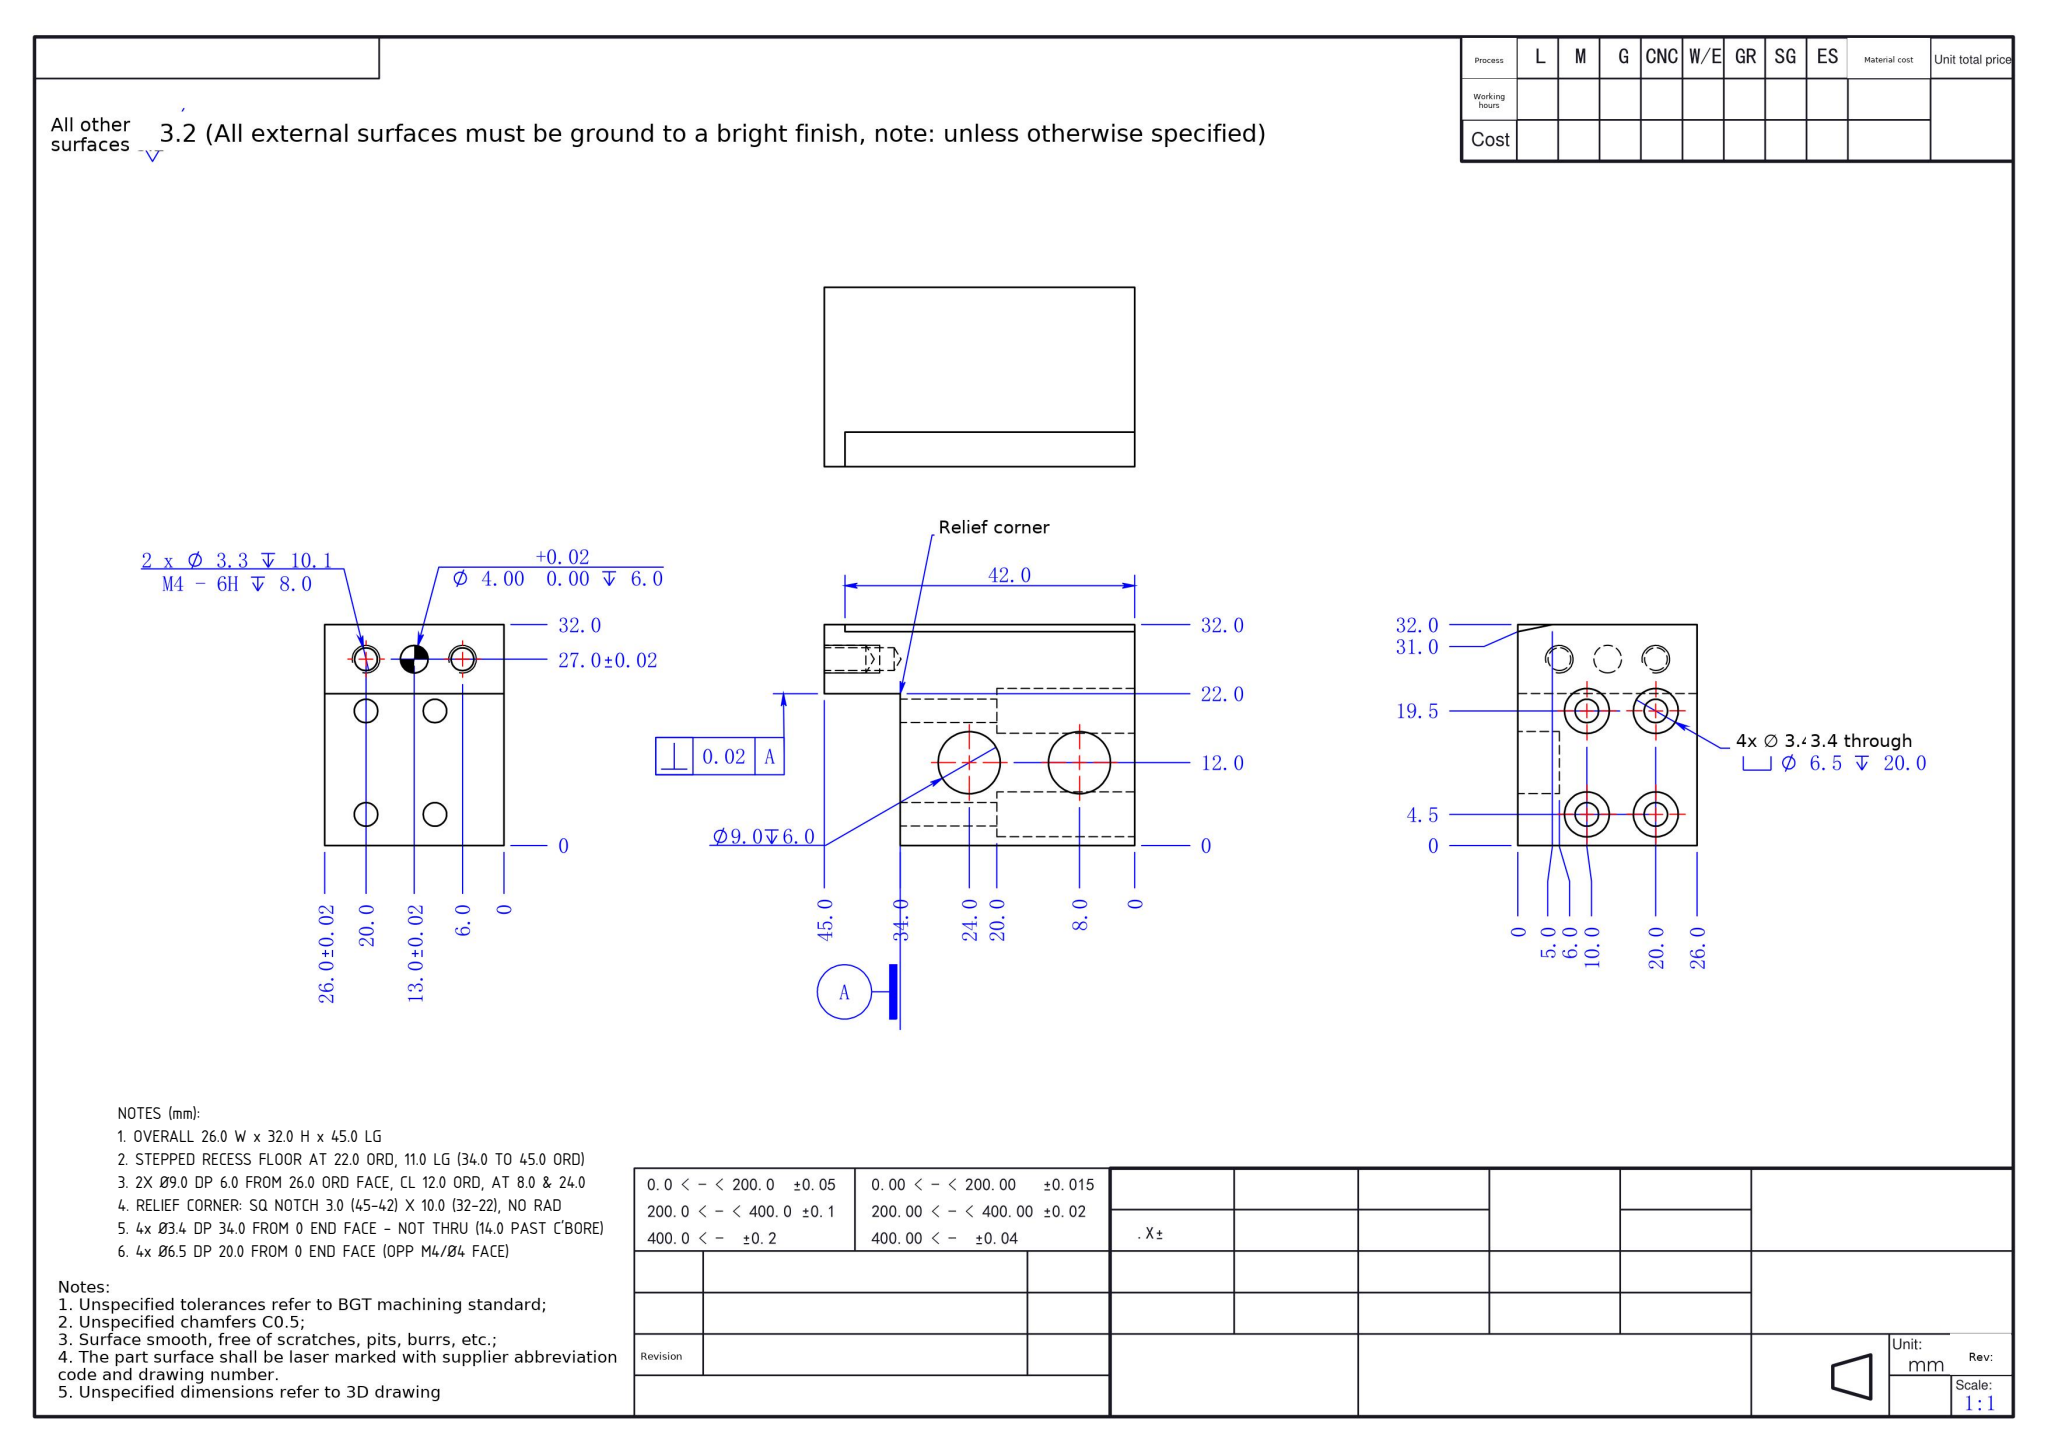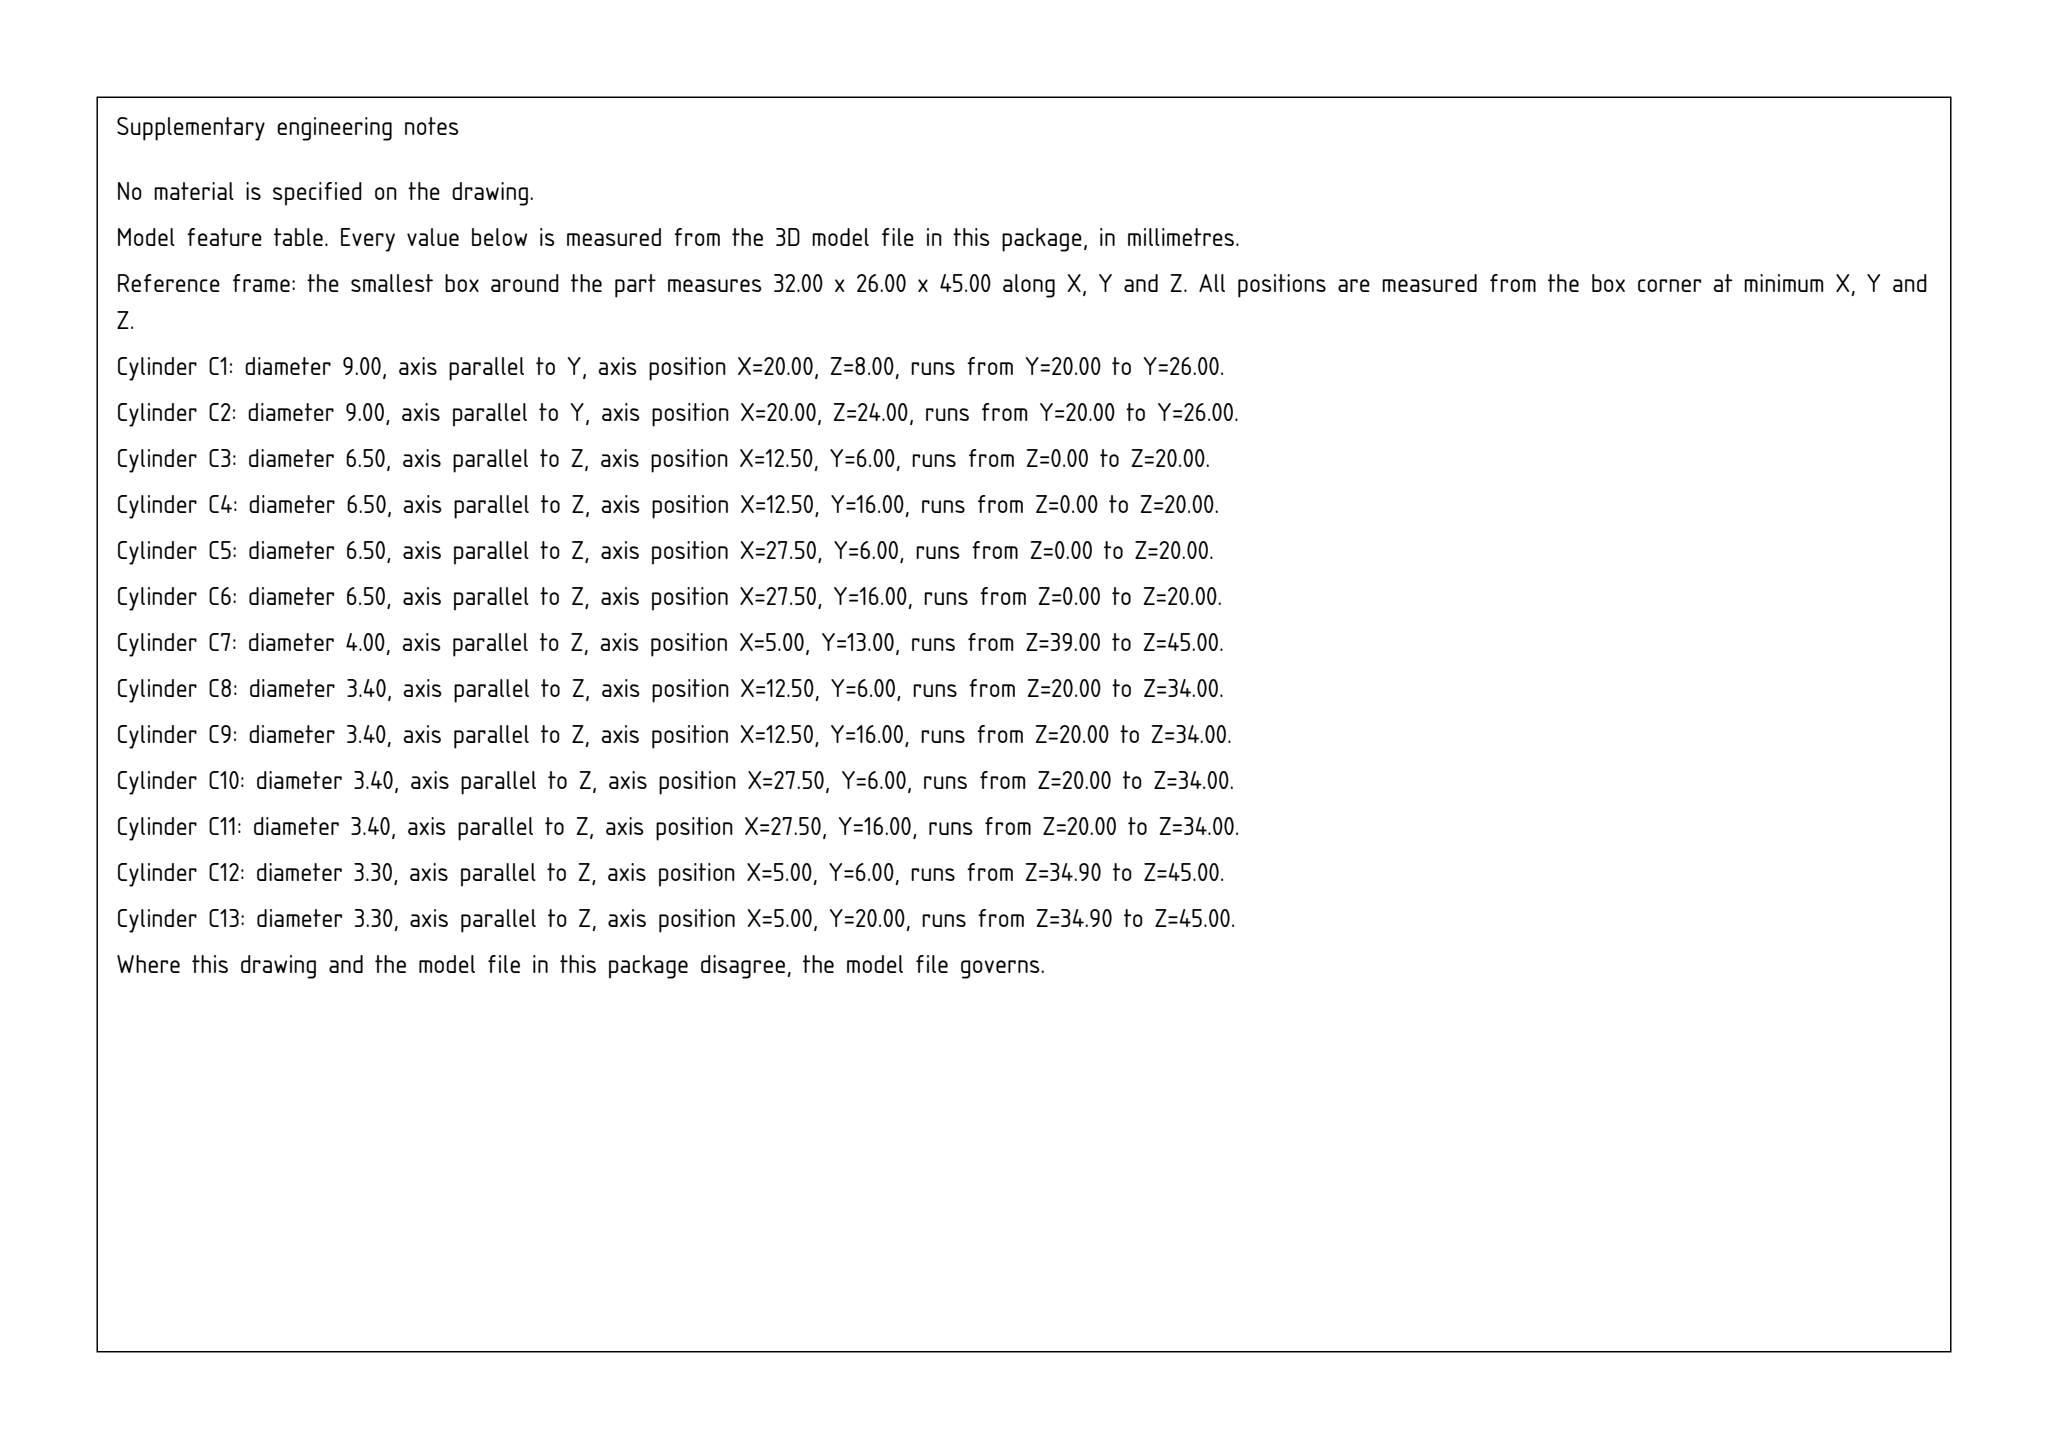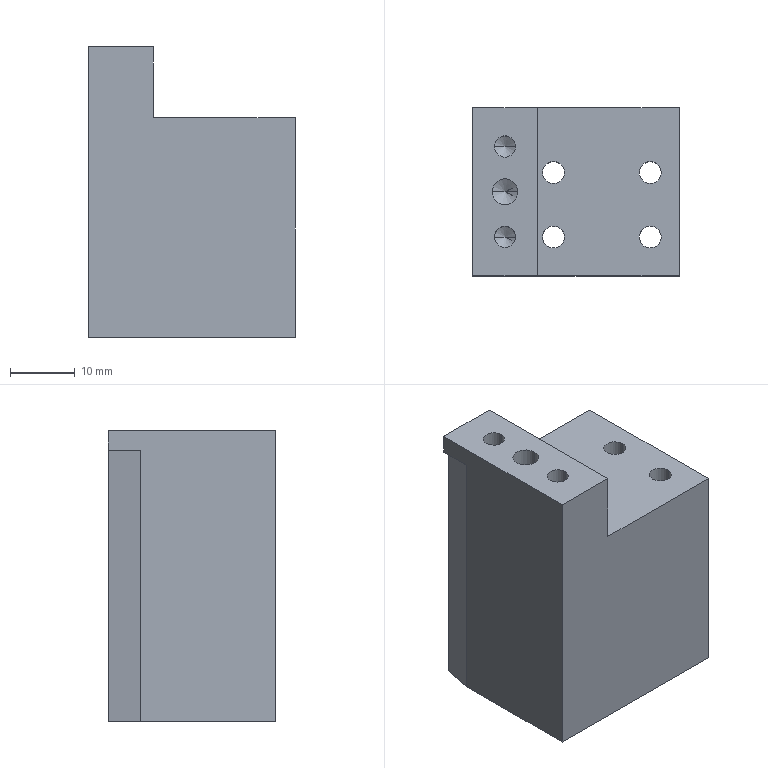Part | SolidWorks | mm | 1 solid | 48 faces | box 32 x 26 x 45 mm | volume 26858 mm3 | cylinder 26 | plane 16 | cone 6 | commonest cylinder face diameters 6.5 x8 3.4 x8 3.3 x4 9 x4 4 x2
Drawing notes:
OVERALL 26.0 W x 32.0 H x 45.0 LG | from the solid: bbox_xyz = [32.0, 26.0, 45.0]
STEPPED RECESS FLOOR AT 22.0 ORD, 11.0 LG (34.0 TO 45.0 ORD) | from the solid: plane x=10.0 (=22.0 ord) is recess floor; z=34.0 to bbox z=45.0 = 11.0 long
2X Ø9.0 DP 6.0 FROM 26.0 ORD FACE, CL 12.0 ORD, AT 8.0 & 24.0 | from the solid: cyl Ø9.0 axis y at x=20 (12.0 ord), z=8.0 & 24.0, len 6.0, end planes y=20.0 x2
RELIEF CORNER: SQ NOTCH 3.0 (45-42) X 10.0 (32-22), NO RAD | from the solid: Z planes at 42.0 and 45.0 with X plane at 10.0 (X0-32 overall); fillet_radii empty = sharp corner
4x Ø3.4 DP 34.0 FROM 0 END FACE - NOT THRU (14.0 PAST C'BORE) | from the solid: Ø3.4 cyls, axis z, length 14.0 below Ø6.5 x 20.0 c'bores: 20.0+14.0=34.0 of 45.0 total Z
4x Ø6.5 DP 20.0 FROM 0 END FACE (OPP M4/Ø4 FACE) | from the solid: Ø6.5 cyls axis z, length 20.0 start at z=0 face; M4 Ø3.3↧10.1 and Ø4↧6.0 start at z=45 face
build123d program:
from build123d import *

# Parameters (mm, degrees)
SKETCH1_W                                       = 35
SKETCH1_H                                       = 26
BOSS_EXTRUDE1_DEPTH                             = 42
SKETCH2_W                                       = 22
SKETCH2_H                                       = 8
CUT_EXTRUDE1_DEPTH                              = 61.539
M3_HEX_SOCKET_HEAD_CAP_SCREW_CBORE1_D           = 3.4
M3_HEX_SOCKET_HEAD_CAP_SCREW_CBORE1_CBORE_D     = 6.5
M3_HEX_SOCKET_HEAD_CAP_SCREW_CBORE1_CBORE_DEPTH = 20
SKETCH5_W                                       = 11
SKETCH5_H                                       = 10
CUT_EXTRUDE2_DEPTH                              = 61.539
SKETCH7_R                                       = 4.5
CUT_EXTRUDE3_DEPTH                              = 6
SKETCH10_W                                      = 1
SKETCH10_H                                      = 32
CUT_EXTRUDE4_DEPTH                              = 61.539
CHAMFER1_SIZE                                   = 3
CHAMFER1_SIZE2                                  = 15
SKETCH13_W                                      = 10
SKETCH13_H                                      = 26
BOSS_EXTRUDE3_DEPTH                             = 3
SKETCH14_W                                      = 2
SKETCH14_H                                      = 26
BOSS_EXTRUDE4_DEPTH                             = 3
M4_TAPPED_HOLE2_D                               = 3.3
M4_TAPPED_HOLE2_DEPTH                           = 10.1
M4_TAPPED_HOLE2_TIP                             = 0.9914
BOSS_EXTRUDE5_DEPTH                             = 10
SKETCH19_W                                      = 2
SKETCH19_H                                      = 26
CUT_EXTRUDE6_DEPTH                              = 63.658
SIZE_MM_DOWEL_PIN_HOLE1_D                       = 4
SIZE_MM_DOWEL_PIN_HOLE1_DEPTH                   = 6
SIZE_MM_DOWEL_PIN_HOLE1_TIP                     = 1.202


with BuildPart() as part:
    # Sketch1 → Boss-Extrude1 (new body)
    with BuildSketch(Plane.XY):
        with Locations((17.5, 13)):
            Rectangle(SKETCH1_W, SKETCH1_H)
    extrude(amount=BOSS_EXTRUDE1_DEPTH)

    # Sketch2 → Cut-Extrude1 (cut, through all)
    with BuildSketch(Plane.XZ):
        with Locations((24, 38)):
            Rectangle(SKETCH2_W, SKETCH2_H)
    extrude(amount=-CUT_EXTRUDE1_DEPTH, mode=Mode.SUBTRACT)

    # M3 Hex Socket Head Cap Screw CBORE1 (through all)
    with Locations(Plane(origin=(0, 0, 0), x_dir=(-1, 0, 0), z_dir=(0, 0, -1))):
        with Locations((-15.5, 16), (-15.5, 6), (-30.5, 16), (-30.5, 6)):
            CounterBoreHole(M3_HEX_SOCKET_HEAD_CAP_SCREW_CBORE1_D / 2, M3_HEX_SOCKET_HEAD_CAP_SCREW_CBORE1_CBORE_D / 2, M3_HEX_SOCKET_HEAD_CAP_SCREW_CBORE1_CBORE_DEPTH)

    # Sketch5 → Cut-Extrude2 (cut, through all)
    with BuildSketch(Plane(origin=(0, 26, 0), x_dir=(1, 0, 0), z_dir=(0, 1, 0))):
        with Locations((5.5, -5)):
            Rectangle(SKETCH5_W, SKETCH5_H)
    extrude(amount=-CUT_EXTRUDE2_DEPTH, mode=Mode.SUBTRACT)

    # Sketch7 → Cut-Extrude3 (cut)
    with BuildSketch(Plane(origin=(0, 26, 0), x_dir=(1, 0, 0), z_dir=(0, 1, 0))):
        with Locations(Location((23, -24, 0), (0, 0, 270))):
            Circle(SKETCH7_R)
        with Locations(Location((23, -8, 0), (0, 0, 270))):
            Circle(SKETCH7_R)
    extrude(amount=-CUT_EXTRUDE3_DEPTH, mode=Mode.SUBTRACT)

    # Sketch10 → Cut-Extrude4 (cut, through all)
    with BuildSketch(Plane(origin=(0, 26, 0), x_dir=(1, 0, 0), z_dir=(0, 1, 0))):
        with Locations((0.5, -26)):
            Rectangle(SKETCH10_W, SKETCH10_H)
    extrude(amount=-CUT_EXTRUDE4_DEPTH, mode=Mode.SUBTRACT)

    # Chamfer1
    chamfer1_edges = [part.edges().sort_by_distance(p)[0] for p in [
        (1, 26, 26),
    ]]
    chamfer1_side = [part.faces().sort_by_distance(p)[0] for p in [
        (17.52, 26, 20.262),
    ]]
    chamfer(chamfer1_edges, length=CHAMFER1_SIZE, length2=CHAMFER1_SIZE2, reference=chamfer1_side[0])

    # Sketch13 → Boss-Extrude3 (add)
    with BuildSketch(Plane.XY.offset(42)):
        with Locations((6, 13)):
            Rectangle(SKETCH13_W, SKETCH13_H)
    extrude(amount=BOSS_EXTRUDE3_DEPTH)

    # Sketch14 → Boss-Extrude4 (add)
    with BuildSketch(Plane.XY.offset(42)):
        with Locations((12, 13)):
            Rectangle(SKETCH14_W, SKETCH14_H)
    extrude(amount=BOSS_EXTRUDE4_DEPTH)

    # M4 Tapped Hole2
    with Locations(Plane.XY.offset(45)):
        with Locations((8, 6), (8, 20)):
            Hole(M4_TAPPED_HOLE2_D / 2, depth=M4_TAPPED_HOLE2_DEPTH)
            with Locations((0, 0, -(M4_TAPPED_HOLE2_DEPTH + M4_TAPPED_HOLE2_TIP / 2))):  # 118° drill point
                Cone(0, M4_TAPPED_HOLE2_D / 2, M4_TAPPED_HOLE2_TIP, mode=Mode.SUBTRACT)

    # Sketch18 → Boss-Extrude5 (add)
    with BuildSketch(Plane(origin=(0, 0, 10), x_dir=(-1, 0, 0), z_dir=(0, 0, -1))):
        Polygon((-1, 0), (-1, 11), (-4, 26), (-11, 26), (-11, 0), align=None)
    extrude(amount=BOSS_EXTRUDE5_DEPTH)

    # Sketch19 → Cut-Extrude6 (cut, through all)
    with BuildSketch(Plane(origin=(0, 0, 0), x_dir=(-1, 0, 0), z_dir=(0, 0, -1))):
        with Locations((-2, 13)):
            Rectangle(SKETCH19_W, SKETCH19_H)
    extrude(amount=-CUT_EXTRUDE6_DEPTH, mode=Mode.SUBTRACT)

    # Size mm Dowel Pin Hole1
    with Locations(Plane.XY.offset(45)):
        with Locations((8, 13)):
            Hole(SIZE_MM_DOWEL_PIN_HOLE1_D / 2, depth=SIZE_MM_DOWEL_PIN_HOLE1_DEPTH)
            with Locations((0, 0, -(SIZE_MM_DOWEL_PIN_HOLE1_DEPTH + SIZE_MM_DOWEL_PIN_HOLE1_TIP / 2))):  # 118° drill point
                Cone(0, SIZE_MM_DOWEL_PIN_HOLE1_D / 2, SIZE_MM_DOWEL_PIN_HOLE1_TIP, mode=Mode.SUBTRACT)


solid = part.part